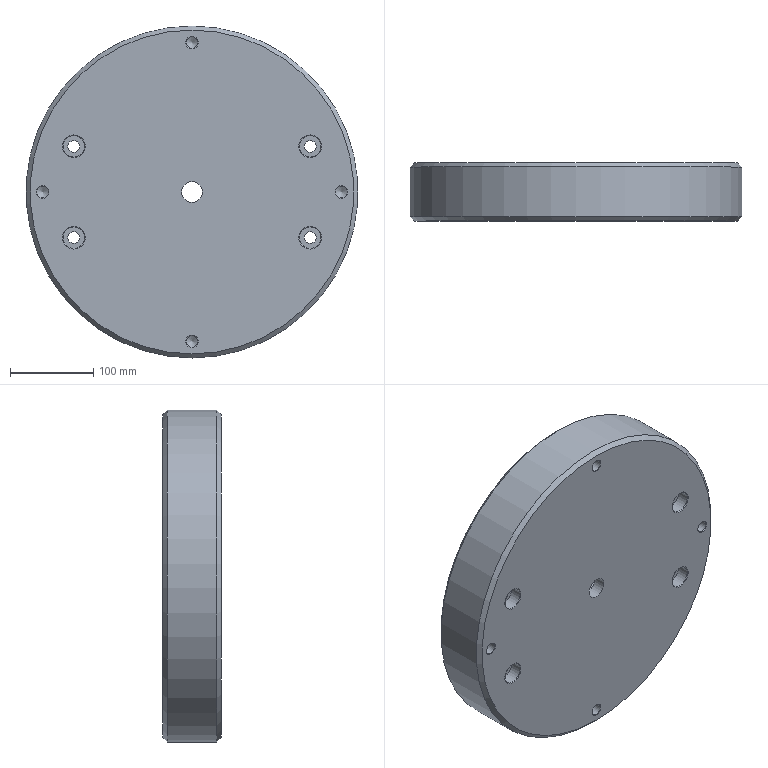Component | NX | DIE_PLATE | 1 solid | 53 faces | volume 8415301 mm3 | cylinder 20 | cone 18 | plane 11 | torus 4 | commonest cylinder face diameters 14 x4 14.2 x4 25.9 x4 6 x4 8 x2 400 x1 25 x1